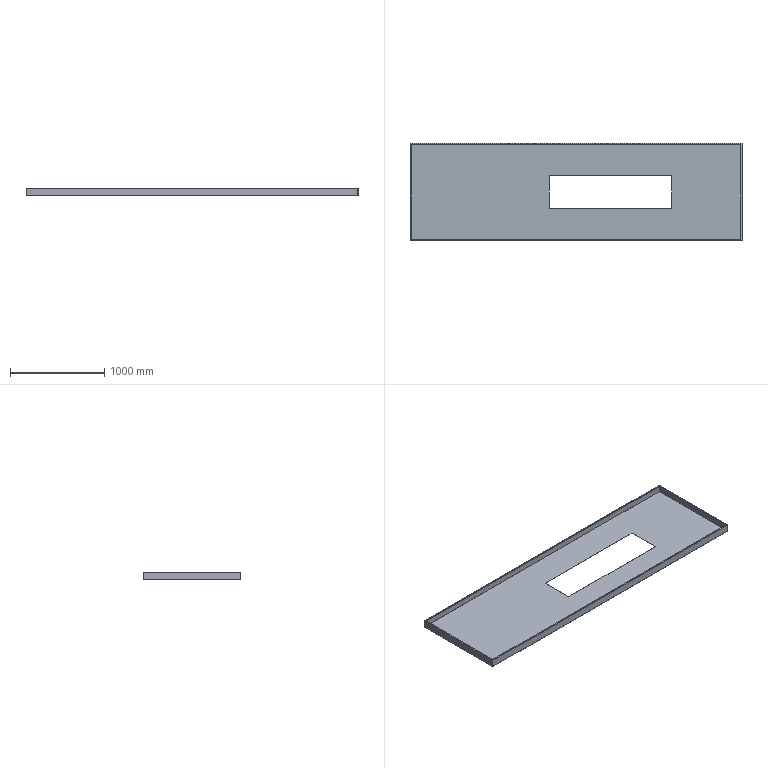Component | NX | DB4_12 | 1 solid | 20 faces | volume 6018762 mm3 | plane 20